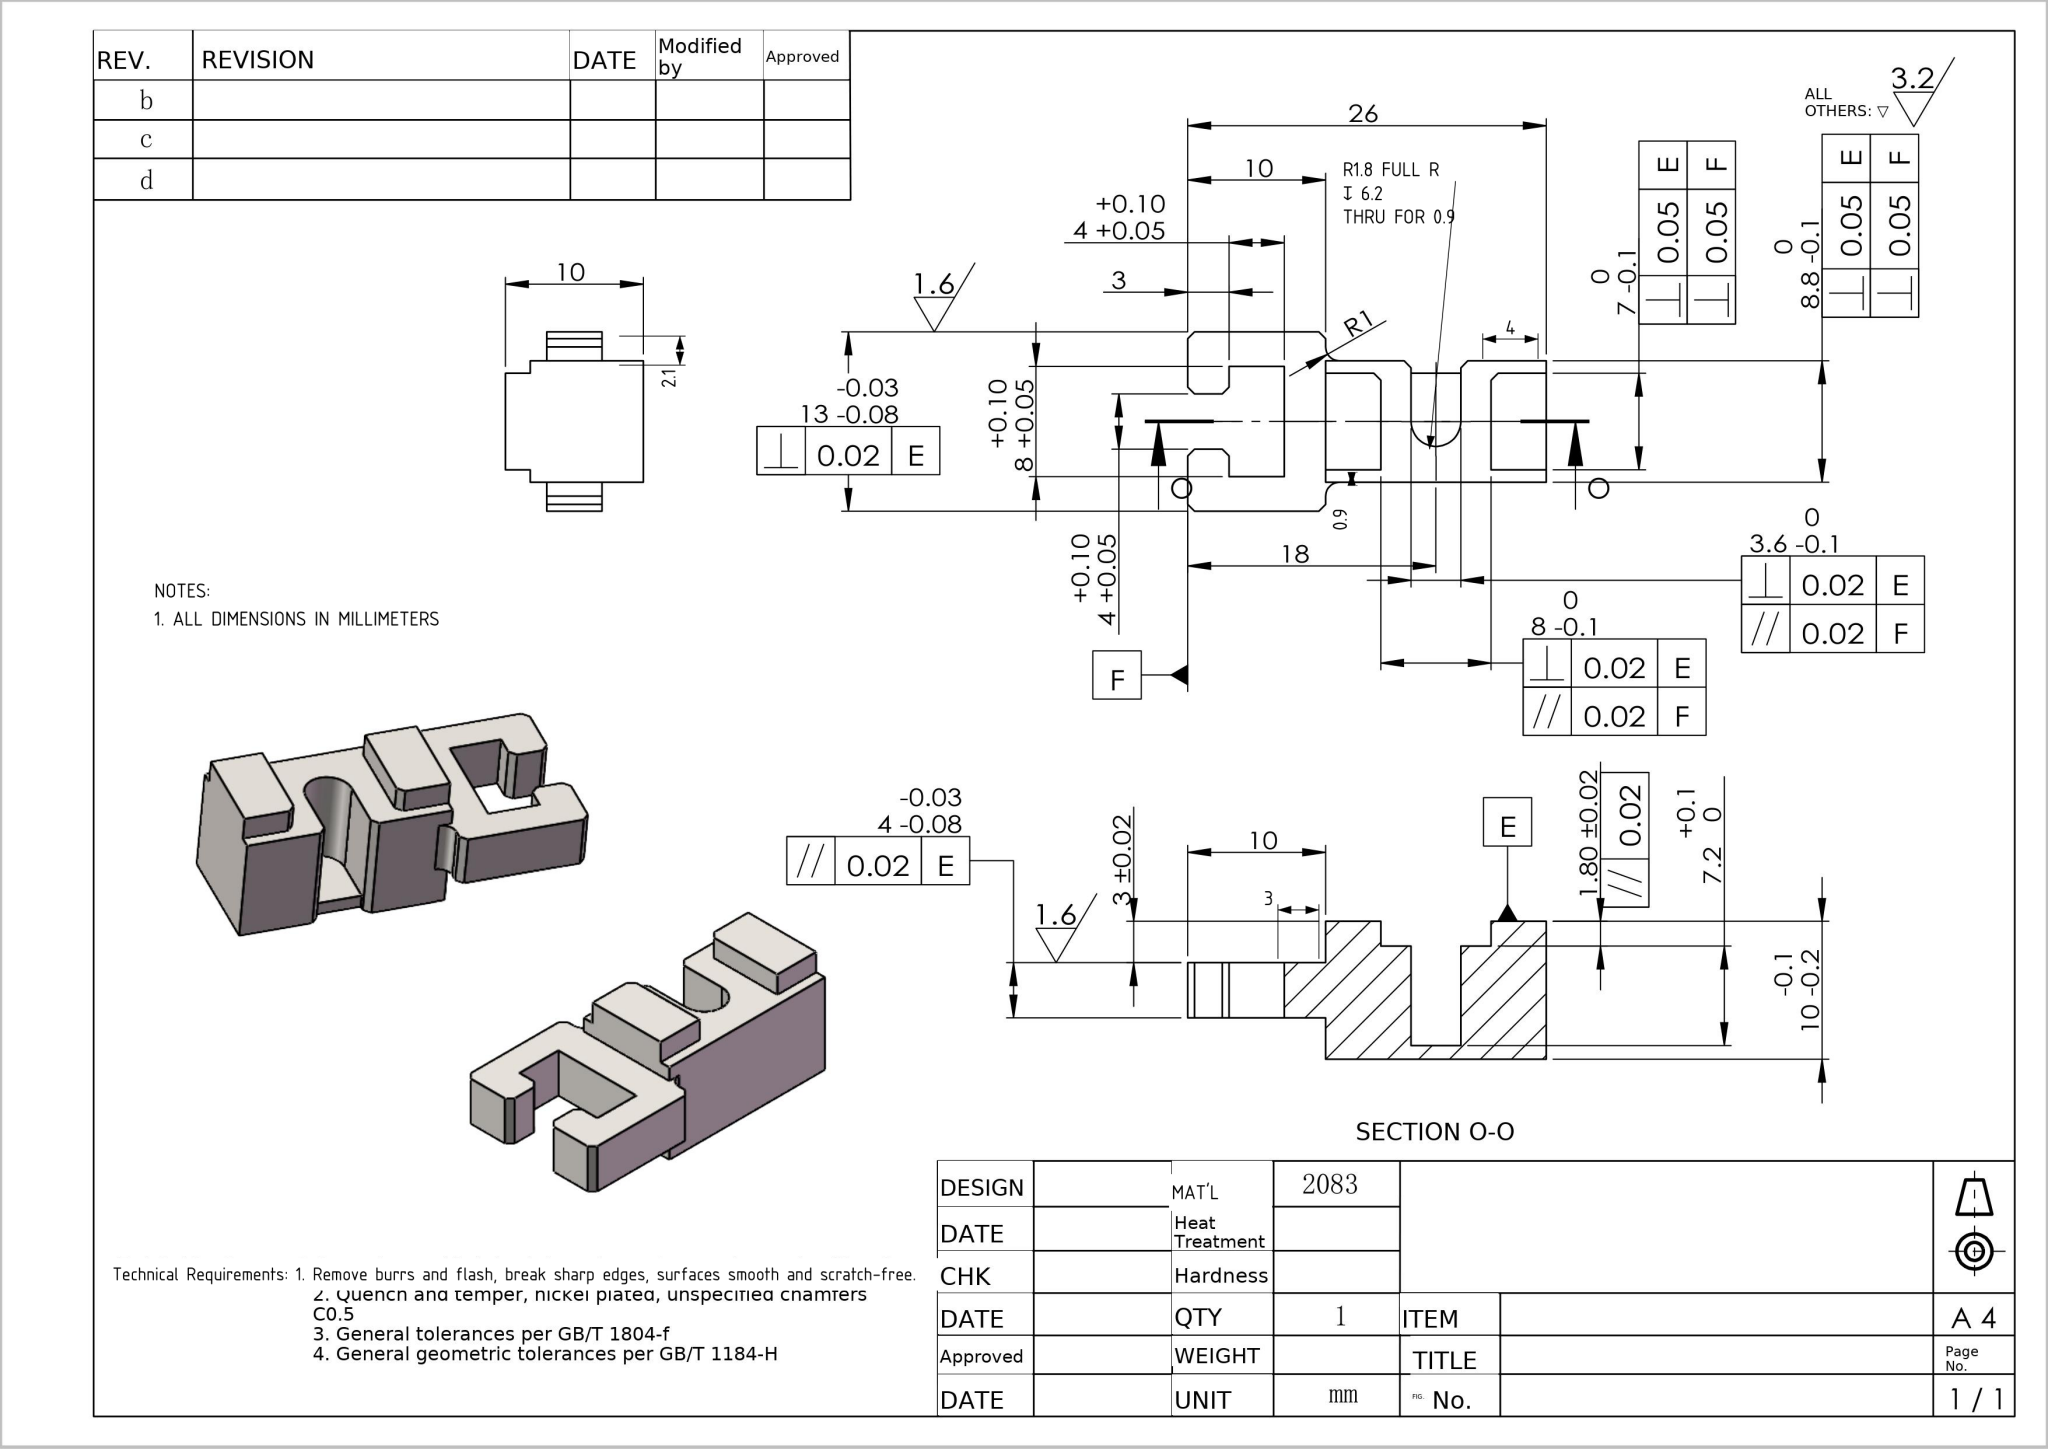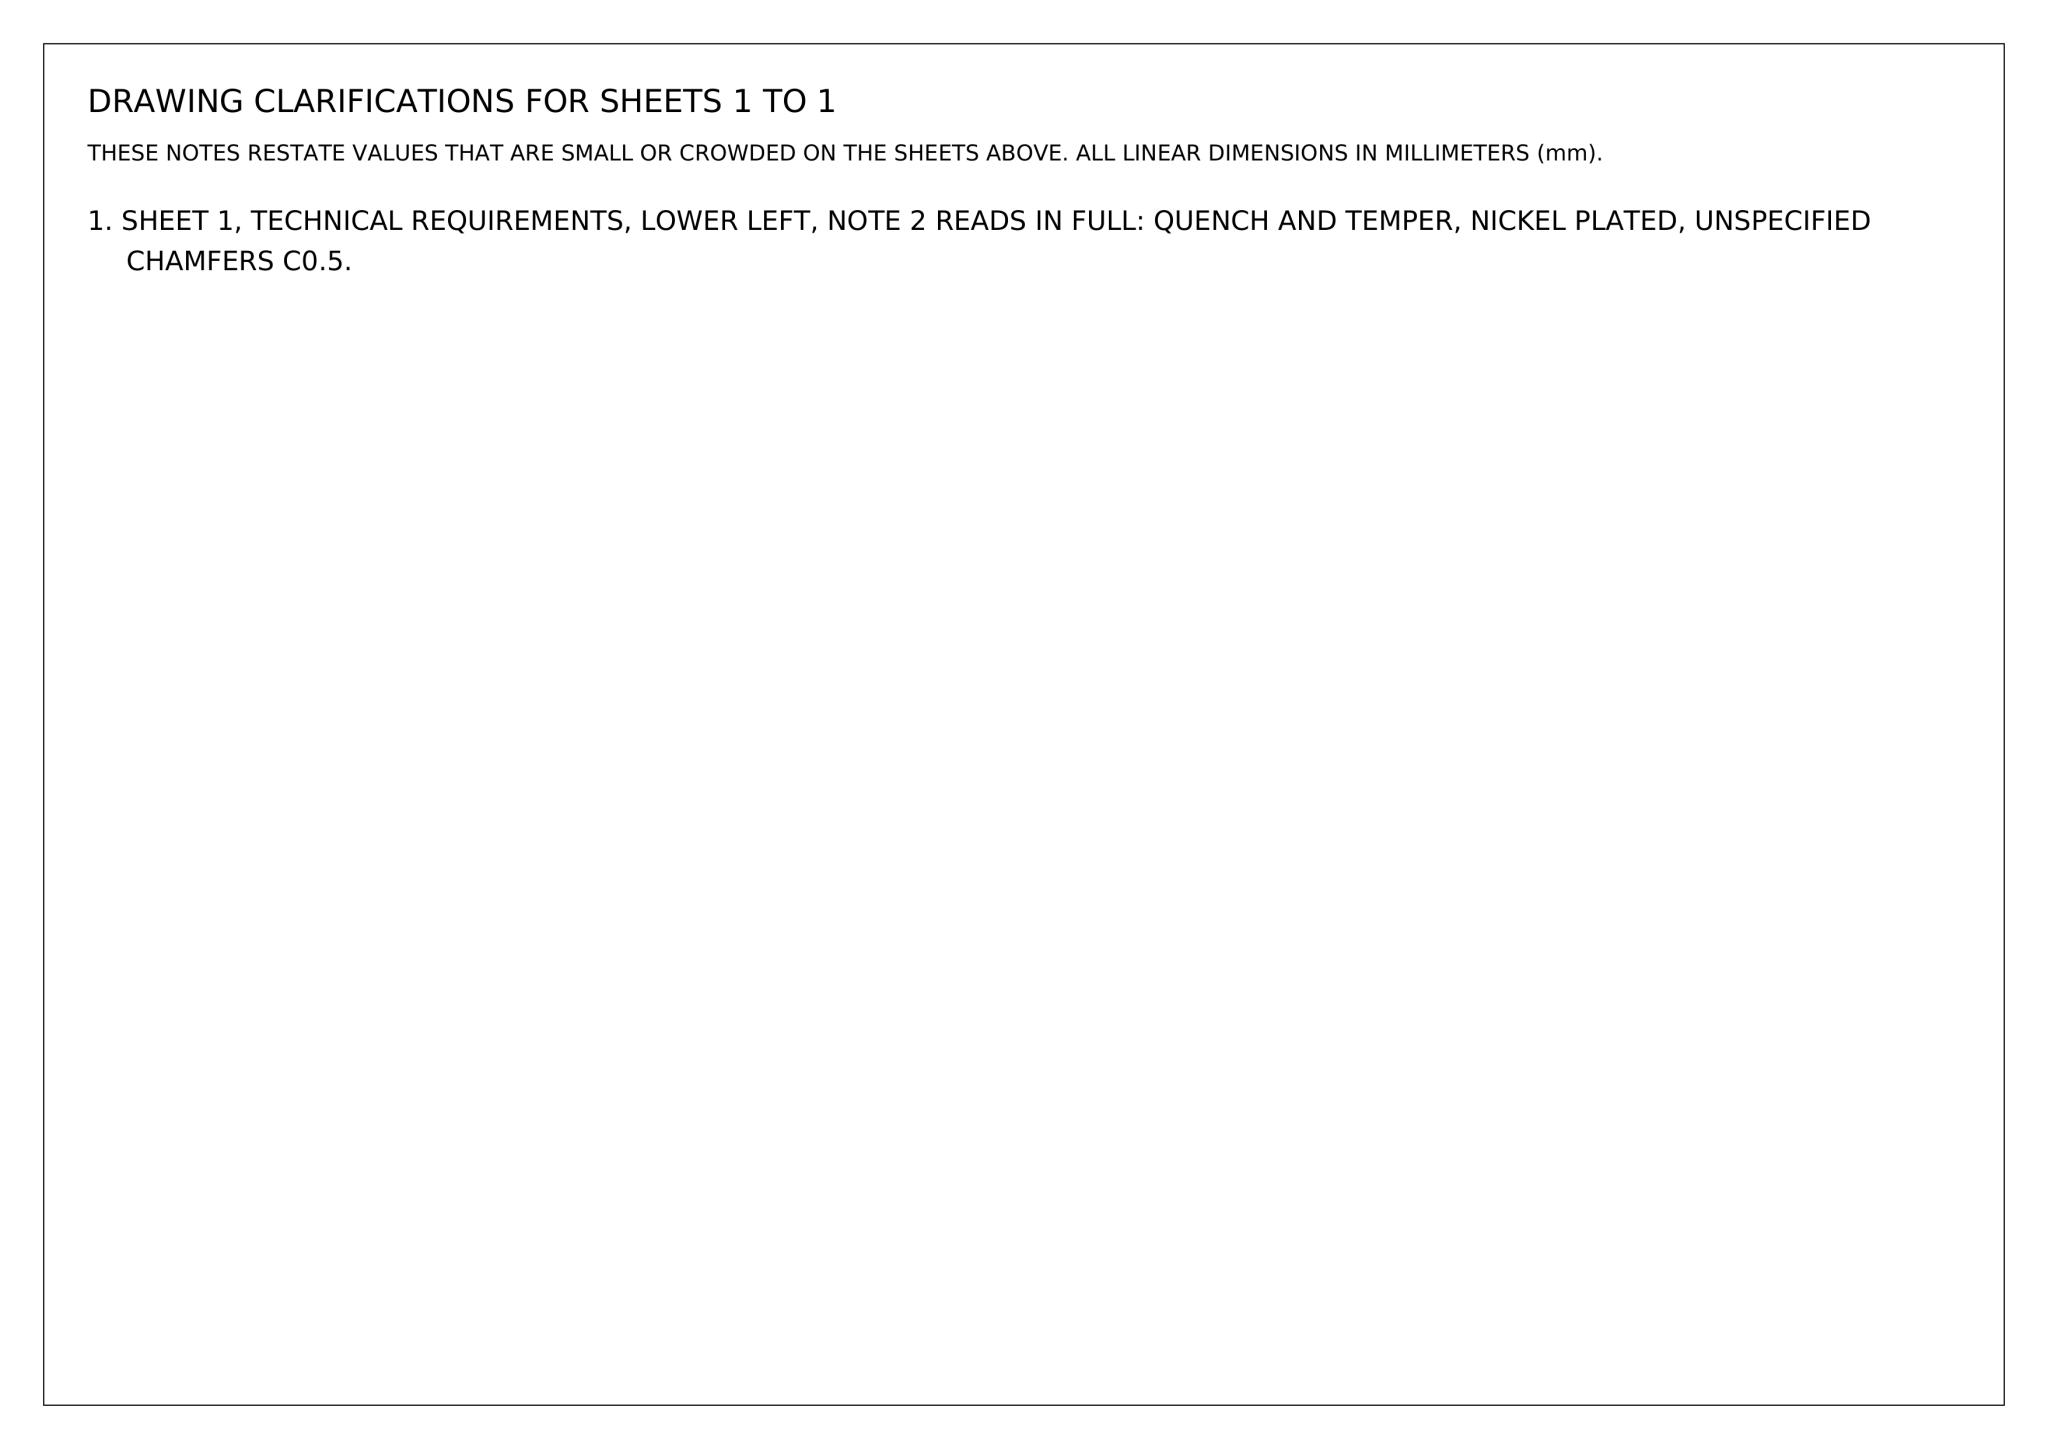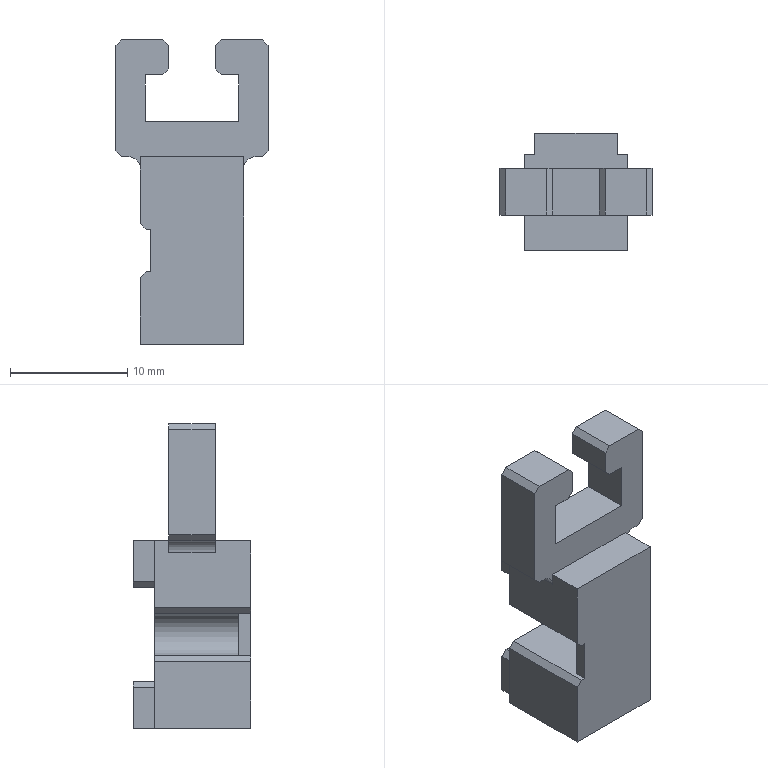Part | NX | mm | Slotted Slide Guide Block 2 | 1 solid | 50 faces | box 13 x 10 x 26 mm | volume 1441 mm3 | plane 47 | cylinder 3 | commonest cylinder face diameters 2 x2 3.6 x1